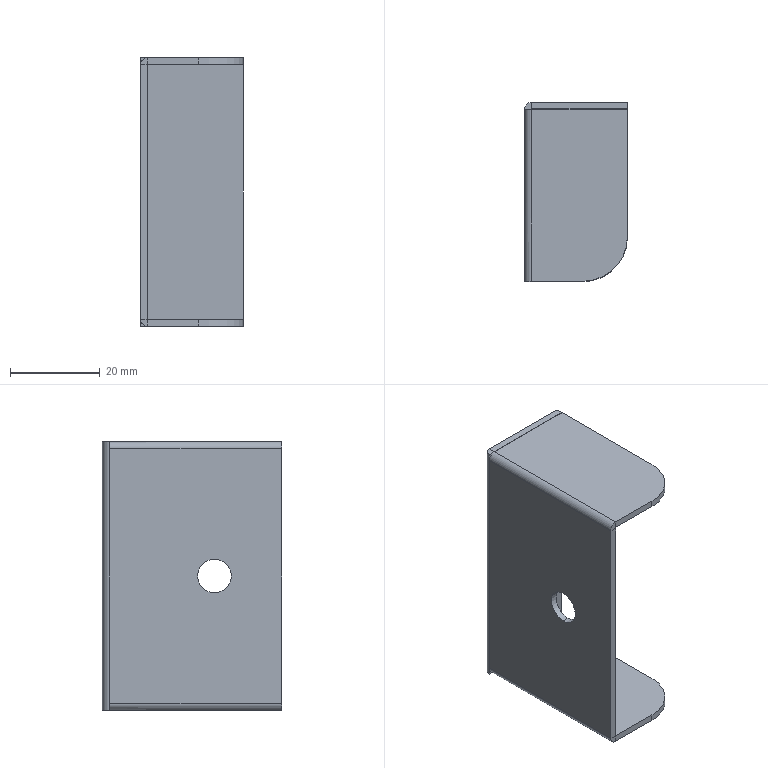Component | SolidWorks | TopPlateWelding-1_AxisFixingPlate2-1 | 1 solid | 37 faces | box 23 x 40 x 60 mm | volume 7806 mm3 | plane 27 | cylinder 10 | commonest cylinder face diameters 0.2 x3 3.2 x3 7.5 x2 20 x2
STEP:
#1=COLOUR_RGB('',0.7922,0.8196,0.9333);
#2=FILL_AREA_STYLE_COLOUR('',#1);
#3=FILL_AREA_STYLE('',(#2));
#4=SURFACE_STYLE_FILL_AREA(#3);
#5=SURFACE_SIDE_STYLE('',(#4));
#6=SURFACE_STYLE_USAGE(.BOTH.,#5);
#7=PRESENTATION_STYLE_ASSIGNMENT((#6));
#8=CARTESIAN_POINT('',(8.937,5.032,15.128));
#9=VERTEX_POINT('',#8);
#10=CARTESIAN_POINT('',(8.937,5.032,14.833));
#11=VERTEX_POINT('',#10);
#12=CARTESIAN_POINT('',(8.937,5.032,14.98));
#13=DIRECTION('',(-1.,-0.,0.));
#14=DIRECTION('',(0.,-1.,0.));
#15=AXIS2_PLACEMENT_3D('',#12,#13,#14);
#16=CIRCLE('',#15,0.1476);
#17=EDGE_CURVE('',#9,#11,#16,.T.);
#18=ORIENTED_EDGE('',*,*,#17,.F.);
#19=CARTESIAN_POINT('',(8.878,5.032,15.128));
#20=VERTEX_POINT('',#19);
#21=CARTESIAN_POINT('',(9.355,5.032,15.128));
#22=DIRECTION('',(-1.,-0.,0.));
#23=VECTOR('',#22,39.37);
#24=LINE('',#21,#23);
#25=EDGE_CURVE('',#9,#20,#24,.T.);
#26=ORIENTED_EDGE('',*,*,#25,.T.);
#27=CARTESIAN_POINT('',(8.878,5.032,14.833));
#28=VERTEX_POINT('',#27);
#29=CARTESIAN_POINT('',(8.878,5.032,14.98));
#30=DIRECTION('',(-1.,-0.,0.));
#31=DIRECTION('',(-0.,0.,-1.));
#32=AXIS2_PLACEMENT_3D('',#29,#30,#31);
#33=CIRCLE('',#32,0.1476);
#34=EDGE_CURVE('',#20,#28,#33,.T.);
#35=ORIENTED_EDGE('',*,*,#34,.T.);
#36=CARTESIAN_POINT('',(9.355,5.032,14.833));
#37=DIRECTION('',(-1.,-0.,0.));
#38=VECTOR('',#37,39.37);
#39=LINE('',#36,#38);
#40=EDGE_CURVE('',#11,#28,#39,.T.);
#41=ORIENTED_EDGE('',*,*,#40,.F.);
#42=EDGE_LOOP('',(#18,#26,#35,#41));
#43=FACE_OUTER_BOUND('',#42,.T.);
#44=CARTESIAN_POINT('',(9.355,5.032,14.98));
#45=DIRECTION('',(-1.,-0.,0.));
#46=DIRECTION('',(-0.,0.,-1.));
#47=AXIS2_PLACEMENT_3D('',#44,#45,#46);
#48=CYLINDRICAL_SURFACE('',#47,0.1476);
#49=ADVANCED_FACE('',(#43),#48,.F.);
#50=CARTESIAN_POINT('',(8.878,5.954,16.161));
#51=VERTEX_POINT('',#50);
#52=CARTESIAN_POINT('',(8.878,5.954,16.098));
#53=VERTEX_POINT('',#52);
#54=CARTESIAN_POINT('',(8.878,5.954,13.799));
#55=DIRECTION('',(-0.,-0.,-1.));
#56=VECTOR('',#55,39.37);
#57=LINE('',#54,#56);
#58=EDGE_CURVE('',#51,#53,#57,.T.);
#59=ORIENTED_EDGE('',*,*,#58,.T.);
#60=CARTESIAN_POINT('',(8.937,5.954,16.161));
#61=VERTEX_POINT('',#60);
#62=CARTESIAN_POINT('',(8.941,5.954,16.098));
#63=DIRECTION('',(-0.,1.,-0.));
#64=DIRECTION('',(0.,0.,-1.));
#65=AXIS2_PLACEMENT_3D('',#62,#63,#64);
#66=CIRCLE('',#65,0.06299);
#67=EDGE_CURVE('',#53,#61,#66,.T.);
#68=ORIENTED_EDGE('',*,*,#67,.T.);
#69=CARTESIAN_POINT('',(8.937,5.954,16.161));
#70=VERTEX_POINT('',#69);
#71=CARTESIAN_POINT('',(8.937,5.954,16.098));
#72=DIRECTION('',(0.,-0.,1.));
#73=VECTOR('',#72,39.37);
#74=LINE('',#71,#73);
#75=EDGE_CURVE('',#61,#70,#74,.T.);
#76=ORIENTED_EDGE('',*,*,#75,.T.);
#77=CARTESIAN_POINT('',(8.937,5.954,16.161));
#78=DIRECTION('',(-1.,-0.,0.));
#79=VECTOR('',#78,39.37);
#80=LINE('',#77,#79);
#81=EDGE_CURVE('',#70,#51,#80,.T.);
#82=ORIENTED_EDGE('',*,*,#81,.T.);
#83=EDGE_LOOP('',(#59,#68,#76,#82));
#84=FACE_OUTER_BOUND('',#83,.T.);
#85=CARTESIAN_POINT('',(8.937,5.954,16.098));
#86=DIRECTION('',(0.,-1.,-0.));
#87=DIRECTION('',(-0.,0.,-1.));
#88=AXIS2_PLACEMENT_3D('',#85,#86,#87);
#89=PLANE('',#88);
#90=ADVANCED_FACE('',(#84),#89,.T.);
#91=CARTESIAN_POINT('',(8.937,5.032,14.98));
#92=DIRECTION('',(-1.,-0.,0.));
#93=DIRECTION('',(0.,-1.,0.));
#94=AXIS2_PLACEMENT_3D('',#91,#92,#93);
#95=CIRCLE('',#94,0.1476);
#96=EDGE_CURVE('',#11,#9,#95,.T.);
#97=ORIENTED_EDGE('',*,*,#96,.T.);
#98=ORIENTED_EDGE('',*,*,#17,.T.);
#99=EDGE_LOOP('',(#97,#98));
#100=FACE_BOUND('',#99,.T.);
#101=CARTESIAN_POINT('',(8.937,5.954,13.862));
#102=VERTEX_POINT('',#101);
#103=CARTESIAN_POINT('',(8.937,5.954,16.098));
#104=VERTEX_POINT('',#103);
#105=CARTESIAN_POINT('',(8.937,5.954,13.799));
#106=DIRECTION('',(0.,0.,1.));
#107=VECTOR('',#106,39.37);
#108=LINE('',#105,#107);
#109=EDGE_CURVE('',#102,#104,#108,.T.);
#110=ORIENTED_EDGE('',*,*,#109,.T.);
#111=CARTESIAN_POINT('',(8.937,4.442,16.098));
#112=VERTEX_POINT('',#111);
#113=CARTESIAN_POINT('',(8.937,4.442,16.098));
#114=DIRECTION('',(-0.,1.,-0.));
#115=VECTOR('',#114,39.37);
#116=LINE('',#113,#115);
#117=EDGE_CURVE('',#112,#104,#116,.T.);
#118=ORIENTED_EDGE('',*,*,#117,.F.);
#119=CARTESIAN_POINT('',(8.937,4.442,13.862));
#120=VERTEX_POINT('',#119);
#121=CARTESIAN_POINT('',(8.937,4.442,13.799));
#122=DIRECTION('',(0.,0.,1.));
#123=VECTOR('',#122,39.37);
#124=LINE('',#121,#123);
#125=EDGE_CURVE('',#120,#112,#124,.T.);
#126=ORIENTED_EDGE('',*,*,#125,.F.);
#127=CARTESIAN_POINT('',(8.937,5.954,13.862));
#128=DIRECTION('',(0.,-1.,0.));
#129=VECTOR('',#128,39.37);
#130=LINE('',#127,#129);
#131=EDGE_CURVE('',#102,#120,#130,.T.);
#132=ORIENTED_EDGE('',*,*,#131,.F.);
#133=EDGE_LOOP('',(#110,#118,#126,#132));
#134=FACE_OUTER_BOUND('',#133,.T.);
#135=CARTESIAN_POINT('',(8.937,4.442,13.799));
#136=DIRECTION('',(1.,0.,-0.));
#137=DIRECTION('',(0.,-1.,0.));
#138=AXIS2_PLACEMENT_3D('',#135,#136,#137);
#139=PLANE('',#138);
#140=ADVANCED_FACE('',(#100,#134),#139,.T.);
#141=CARTESIAN_POINT('',(8.878,5.032,14.98));
#142=DIRECTION('',(-1.,-0.,0.));
#143=DIRECTION('',(-0.,0.,-1.));
#144=AXIS2_PLACEMENT_3D('',#141,#142,#143);
#145=CIRCLE('',#144,0.1476);
#146=EDGE_CURVE('',#28,#20,#145,.T.);
#147=ORIENTED_EDGE('',*,*,#146,.F.);
#148=ORIENTED_EDGE('',*,*,#34,.F.);
#149=EDGE_LOOP('',(#147,#148));
#150=FACE_BOUND('',#149,.T.);
#151=CARTESIAN_POINT('',(8.878,4.442,16.098));
#152=VERTEX_POINT('',#151);
#153=CARTESIAN_POINT('',(8.878,4.442,16.098));
#154=DIRECTION('',(-0.,1.,-0.));
#155=VECTOR('',#154,39.37);
#156=LINE('',#153,#155);
#157=EDGE_CURVE('',#152,#53,#156,.T.);
#158=ORIENTED_EDGE('',*,*,#157,.T.);
#159=CARTESIAN_POINT('',(8.878,5.954,13.862));
#160=VERTEX_POINT('',#159);
#161=CARTESIAN_POINT('',(8.878,5.954,13.799));
#162=DIRECTION('',(0.,0.,1.));
#163=VECTOR('',#162,39.37);
#164=LINE('',#161,#163);
#165=EDGE_CURVE('',#160,#53,#164,.T.);
#166=ORIENTED_EDGE('',*,*,#165,.F.);
#167=CARTESIAN_POINT('',(8.878,4.442,13.862));
#168=VERTEX_POINT('',#167);
#169=CARTESIAN_POINT('',(8.878,5.954,13.862));
#170=DIRECTION('',(0.,-1.,0.));
#171=VECTOR('',#170,39.37);
#172=LINE('',#169,#171);
#173=EDGE_CURVE('',#160,#168,#172,.T.);
#174=ORIENTED_EDGE('',*,*,#173,.T.);
#175=CARTESIAN_POINT('',(8.878,4.442,13.799));
#176=DIRECTION('',(0.,0.,1.));
#177=VECTOR('',#176,39.37);
#178=LINE('',#175,#177);
#179=EDGE_CURVE('',#168,#152,#178,.T.);
#180=ORIENTED_EDGE('',*,*,#179,.T.);
#181=EDGE_LOOP('',(#158,#166,#174,#180));
#182=FACE_OUTER_BOUND('',#181,.T.);
#183=CARTESIAN_POINT('',(8.878,4.442,13.799));
#184=DIRECTION('',(1.,0.,-0.));
#185=DIRECTION('',(0.,-1.,0.));
#186=AXIS2_PLACEMENT_3D('',#183,#184,#185);
#187=PLANE('',#186);
#188=ADVANCED_FACE('',(#150,#182),#187,.F.);
#189=ORIENTED_EDGE('',*,*,#125,.T.);
#190=CARTESIAN_POINT('',(8.937,4.442,16.098));
#191=DIRECTION('',(-1.,-0.,0.));
#192=VECTOR('',#191,39.37);
#193=LINE('',#190,#192);
#194=EDGE_CURVE('',#112,#152,#193,.T.);
#195=ORIENTED_EDGE('',*,*,#194,.T.);
#196=ORIENTED_EDGE('',*,*,#179,.F.);
#197=CARTESIAN_POINT('',(8.937,4.442,13.862));
#198=DIRECTION('',(-1.,-0.,0.));
#199=VECTOR('',#198,39.37);
#200=LINE('',#197,#199);
#201=EDGE_CURVE('',#120,#168,#200,.T.);
#202=ORIENTED_EDGE('',*,*,#201,.F.);
#203=EDGE_LOOP('',(#189,#195,#196,#202));
#204=FACE_OUTER_BOUND('',#203,.T.);
#205=CARTESIAN_POINT('',(8.878,4.442,13.799));
#206=DIRECTION('',(0.,-1.,0.));
#207=DIRECTION('',(-0.,-0.,-1.));
#208=AXIS2_PLACEMENT_3D('',#205,#206,#207);
#209=PLANE('',#208);
#210=ADVANCED_FACE('',(#204),#209,.T.);
#211=CARTESIAN_POINT('',(8.937,5.954,13.799));
#212=VERTEX_POINT('',#211);
#213=CARTESIAN_POINT('',(8.937,5.954,13.799));
#214=VERTEX_POINT('',#213);
#215=CARTESIAN_POINT('',(8.937,5.954,13.799));
#216=DIRECTION('',(0.,0.,1.));
#217=VECTOR('',#216,39.37);
#218=LINE('',#215,#217);
#219=EDGE_CURVE('',#212,#214,#218,.T.);
#220=ORIENTED_EDGE('',*,*,#219,.T.);
#221=CARTESIAN_POINT('',(8.941,5.954,13.862));
#222=DIRECTION('',(-0.,1.,-0.));
#223=DIRECTION('',(0.,0.,1.));
#224=AXIS2_PLACEMENT_3D('',#221,#222,#223);
#225=CIRCLE('',#224,0.06299);
#226=EDGE_CURVE('',#214,#160,#225,.T.);
#227=ORIENTED_EDGE('',*,*,#226,.T.);
#228=CARTESIAN_POINT('',(8.878,5.954,13.799));
#229=VERTEX_POINT('',#228);
#230=CARTESIAN_POINT('',(8.878,5.954,13.799));
#231=DIRECTION('',(0.,0.,1.));
#232=VECTOR('',#231,39.37);
#233=LINE('',#230,#232);
#234=EDGE_CURVE('',#229,#160,#233,.T.);
#235=ORIENTED_EDGE('',*,*,#234,.F.);
#236=CARTESIAN_POINT('',(8.878,5.954,13.799));
#237=DIRECTION('',(1.,0.,-0.));
#238=VECTOR('',#237,39.37);
#239=LINE('',#236,#238);
#240=EDGE_CURVE('',#229,#212,#239,.T.);
#241=ORIENTED_EDGE('',*,*,#240,.T.);
#242=EDGE_LOOP('',(#220,#227,#235,#241));
#243=FACE_OUTER_BOUND('',#242,.T.);
#244=CARTESIAN_POINT('',(8.937,5.954,13.799));
#245=DIRECTION('',(0.,-1.,0.));
#246=DIRECTION('',(-0.,-0.,-1.));
#247=AXIS2_PLACEMENT_3D('',#244,#245,#246);
#248=PLANE('',#247);
#249=ADVANCED_FACE('',(#243),#248,.T.);
#250=ORIENTED_EDGE('',*,*,#240,.F.);
#251=CARTESIAN_POINT('',(8.941,6.017,13.799));
#252=VERTEX_POINT('',#251);
#253=CARTESIAN_POINT('',(8.941,5.954,13.799));
#254=DIRECTION('',(-0.,-0.,-1.));
#255=DIRECTION('',(-1.,0.,0.));
#256=AXIS2_PLACEMENT_3D('',#253,#254,#255);
#257=CIRCLE('',#256,0.06299);
#258=EDGE_CURVE('',#229,#252,#257,.T.);
#259=ORIENTED_EDGE('',*,*,#258,.T.);
#260=CARTESIAN_POINT('',(8.941,5.958,13.799));
#261=VERTEX_POINT('',#260);
#262=CARTESIAN_POINT('',(8.941,5.958,13.799));
#263=DIRECTION('',(-0.,1.,-0.));
#264=VECTOR('',#263,39.37);
#265=LINE('',#262,#264);
#266=EDGE_CURVE('',#261,#252,#265,.T.);
#267=ORIENTED_EDGE('',*,*,#266,.F.);
#268=CARTESIAN_POINT('',(8.941,5.954,13.799));
#269=DIRECTION('',(-0.,-0.,-1.));
#270=DIRECTION('',(1.,0.,0.));
#271=AXIS2_PLACEMENT_3D('',#268,#269,#270);
#272=CIRCLE('',#271,0.003937);
#273=EDGE_CURVE('',#212,#261,#272,.T.);
#274=ORIENTED_EDGE('',*,*,#273,.F.);
#275=EDGE_LOOP('',(#250,#259,#267,#274));
#276=FACE_OUTER_BOUND('',#275,.T.);
#277=CARTESIAN_POINT('',(8.878,5.954,13.799));
#278=DIRECTION('',(-0.,-0.,-1.));
#279=DIRECTION('',(1.,0.,-0.));
#280=AXIS2_PLACEMENT_3D('',#277,#278,#279);
#281=PLANE('',#280);
#282=ADVANCED_FACE('',(#276),#281,.T.);
#283=CARTESIAN_POINT('',(8.941,6.017,16.161));
#284=VERTEX_POINT('',#283);
#285=CARTESIAN_POINT('',(8.941,5.958,16.161));
#286=VERTEX_POINT('',#285);
#287=CARTESIAN_POINT('',(8.941,6.017,16.161));
#288=DIRECTION('',(0.,-1.,0.));
#289=VECTOR('',#288,39.37);
#290=LINE('',#287,#289);
#291=EDGE_CURVE('',#284,#286,#290,.T.);
#292=ORIENTED_EDGE('',*,*,#291,.F.);
#293=CARTESIAN_POINT('',(8.941,5.954,16.161));
#294=DIRECTION('',(-0.,-0.,-1.));
#295=DIRECTION('',(-1.,0.,0.));
#296=AXIS2_PLACEMENT_3D('',#293,#294,#295);
#297=CIRCLE('',#296,0.06299);
#298=EDGE_CURVE('',#51,#284,#297,.T.);
#299=ORIENTED_EDGE('',*,*,#298,.F.);
#300=ORIENTED_EDGE('',*,*,#81,.F.);
#301=CARTESIAN_POINT('',(8.941,5.954,16.161));
#302=DIRECTION('',(-0.,-0.,-1.));
#303=DIRECTION('',(1.,0.,0.));
#304=AXIS2_PLACEMENT_3D('',#301,#302,#303);
#305=CIRCLE('',#304,0.003937);
#306=EDGE_CURVE('',#70,#286,#305,.T.);
#307=ORIENTED_EDGE('',*,*,#306,.T.);
#308=EDGE_LOOP('',(#292,#299,#300,#307));
#309=FACE_OUTER_BOUND('',#308,.T.);
#310=CARTESIAN_POINT('',(8.941,6.017,16.161));
#311=DIRECTION('',(0.,0.,1.));
#312=DIRECTION('',(-1.,-0.,0.));
#313=AXIS2_PLACEMENT_3D('',#310,#311,#312);
#314=PLANE('',#313);
#315=ADVANCED_FACE('',(#309),#314,.T.);
#316=CARTESIAN_POINT('',(9.783,5.958,16.161));
#317=VERTEX_POINT('',#316);
#318=CARTESIAN_POINT('',(9.783,6.011,16.161));
#319=VERTEX_POINT('',#318);
#320=CARTESIAN_POINT('',(9.783,5.958,16.161));
#321=DIRECTION('',(-0.,1.,-0.));
#322=VECTOR('',#321,39.37);
#323=LINE('',#320,#322);
#324=EDGE_CURVE('',#317,#319,#323,.T.);
#325=ORIENTED_EDGE('',*,*,#324,.T.);
#326=CARTESIAN_POINT('',(9.778,6.017,16.161));
#327=VERTEX_POINT('',#326);
#328=CARTESIAN_POINT('',(9.389,6.405,16.161));
#329=DIRECTION('',(-0.7071,0.7071,0.));
#330=VECTOR('',#329,39.37);
#331=LINE('',#328,#330);
#332=EDGE_CURVE('',#319,#327,#331,.T.);
#333=ORIENTED_EDGE('',*,*,#332,.T.);
#334=CARTESIAN_POINT('',(8.878,6.017,16.161));
#335=DIRECTION('',(1.,0.,-0.));
#336=VECTOR('',#335,39.37);
#337=LINE('',#334,#336);
#338=EDGE_CURVE('',#284,#327,#337,.T.);
#339=ORIENTED_EDGE('',*,*,#338,.F.);
#340=ORIENTED_EDGE('',*,*,#291,.T.);
#341=CARTESIAN_POINT('',(8.878,5.958,16.161));
#342=DIRECTION('',(1.,0.,-0.));
#343=VECTOR('',#342,39.37);
#344=LINE('',#341,#343);
#345=EDGE_CURVE('',#286,#317,#344,.T.);
#346=ORIENTED_EDGE('',*,*,#345,.T.);
#347=EDGE_LOOP('',(#325,#333,#339,#340,#346));
#348=FACE_OUTER_BOUND('',#347,.T.);
#349=CARTESIAN_POINT('',(8.937,5.954,16.161));
#350=DIRECTION('',(0.,0.,1.));
#351=DIRECTION('',(-1.,-0.,0.));
#352=AXIS2_PLACEMENT_3D('',#349,#350,#351);
#353=PLANE('',#352);
#354=ADVANCED_FACE('',(#348),#353,.T.);
#355=ORIENTED_EDGE('',*,*,#338,.T.);
#356=CARTESIAN_POINT('',(9.778,6.017,13.799));
#357=VERTEX_POINT('',#356);
#358=CARTESIAN_POINT('',(9.778,6.017,13.799));
#359=DIRECTION('',(-0.,-0.,-1.));
#360=VECTOR('',#359,39.37);
#361=LINE('',#358,#360);
#362=EDGE_CURVE('',#327,#357,#361,.T.);
#363=ORIENTED_EDGE('',*,*,#362,.T.);
#364=CARTESIAN_POINT('',(8.878,6.017,13.799));
#365=DIRECTION('',(1.,0.,-0.));
#366=VECTOR('',#365,39.37);
#367=LINE('',#364,#366);
#368=EDGE_CURVE('',#252,#357,#367,.T.);
#369=ORIENTED_EDGE('',*,*,#368,.F.);
#370=CARTESIAN_POINT('',(8.941,6.017,13.799));
#371=DIRECTION('',(0.,0.,1.));
#372=VECTOR('',#371,39.37);
#373=LINE('',#370,#372);
#374=EDGE_CURVE('',#252,#284,#373,.T.);
#375=ORIENTED_EDGE('',*,*,#374,.T.);
#376=EDGE_LOOP('',(#355,#363,#369,#375));
#377=FACE_OUTER_BOUND('',#376,.T.);
#378=CARTESIAN_POINT('',(8.878,6.017,13.799));
#379=DIRECTION('',(0.,-1.,0.));
#380=DIRECTION('',(-0.,-0.,-1.));
#381=AXIS2_PLACEMENT_3D('',#378,#379,#380);
#382=PLANE('',#381);
#383=ADVANCED_FACE('',(#377),#382,.F.);
#384=CARTESIAN_POINT('',(9.783,5.958,13.799));
#385=VERTEX_POINT('',#384);
#386=CARTESIAN_POINT('',(9.783,6.011,13.799));
#387=VERTEX_POINT('',#386);
#388=CARTESIAN_POINT('',(9.783,5.958,13.799));
#389=DIRECTION('',(-0.,1.,-0.));
#390=VECTOR('',#389,39.37);
#391=LINE('',#388,#390);
#392=EDGE_CURVE('',#385,#387,#391,.T.);
#393=ORIENTED_EDGE('',*,*,#392,.T.);
#394=CARTESIAN_POINT('',(9.783,6.011,16.161));
#395=DIRECTION('',(0.,0.,1.));
#396=VECTOR('',#395,39.37);
#397=LINE('',#394,#396);
#398=EDGE_CURVE('',#387,#319,#397,.T.);
#399=ORIENTED_EDGE('',*,*,#398,.T.);
#400=ORIENTED_EDGE('',*,*,#324,.F.);
#401=CARTESIAN_POINT('',(9.783,5.958,13.799));
#402=DIRECTION('',(0.,0.,1.));
#403=VECTOR('',#402,39.37);
#404=LINE('',#401,#403);
#405=EDGE_CURVE('',#385,#317,#404,.T.);
#406=ORIENTED_EDGE('',*,*,#405,.F.);
#407=EDGE_LOOP('',(#393,#399,#400,#406));
#408=FACE_OUTER_BOUND('',#407,.T.);
#409=CARTESIAN_POINT('',(9.783,5.958,13.799));
#410=DIRECTION('',(1.,0.,-0.));
#411=DIRECTION('',(0.,0.,1.));
#412=AXIS2_PLACEMENT_3D('',#409,#410,#411);
#413=PLANE('',#412);
#414=ADVANCED_FACE('',(#408),#413,.T.);
#415=ORIENTED_EDGE('',*,*,#345,.F.);
#416=CARTESIAN_POINT('',(8.941,5.958,13.799));
#417=DIRECTION('',(0.,0.,1.));
#418=VECTOR('',#417,39.37);
#419=LINE('',#416,#418);
#420=EDGE_CURVE('',#261,#286,#419,.T.);
#421=ORIENTED_EDGE('',*,*,#420,.F.);
#422=CARTESIAN_POINT('',(8.878,5.958,13.799));
#423=DIRECTION('',(1.,0.,-0.));
#424=VECTOR('',#423,39.37);
#425=LINE('',#422,#424);
#426=EDGE_CURVE('',#261,#385,#425,.T.);
#427=ORIENTED_EDGE('',*,*,#426,.T.);
#428=ORIENTED_EDGE('',*,*,#405,.T.);
#429=EDGE_LOOP('',(#415,#421,#427,#428));
#430=FACE_OUTER_BOUND('',#429,.T.);
#431=CARTESIAN_POINT('',(8.878,5.958,13.799));
#432=DIRECTION('',(0.,-1.,0.));
#433=DIRECTION('',(-0.,-0.,-1.));
#434=AXIS2_PLACEMENT_3D('',#431,#432,#433);
#435=PLANE('',#434);
#436=ADVANCED_FACE('',(#430),#435,.T.);
#437=ORIENTED_EDGE('',*,*,#306,.F.);
#438=ORIENTED_EDGE('',*,*,#75,.F.);
#439=CARTESIAN_POINT('',(8.937,5.954,16.098));
#440=DIRECTION('',(0.,-0.,1.));
#441=VECTOR('',#440,39.37);
#442=LINE('',#439,#441);
#443=EDGE_CURVE('',#104,#61,#442,.T.);
#444=ORIENTED_EDGE('',*,*,#443,.F.);
#445=ORIENTED_EDGE('',*,*,#109,.F.);
#446=CARTESIAN_POINT('',(8.937,5.954,13.799));
#447=DIRECTION('',(0.,0.,1.));
#448=VECTOR('',#447,39.37);
#449=LINE('',#446,#448);
#450=EDGE_CURVE('',#214,#102,#449,.T.);
#451=ORIENTED_EDGE('',*,*,#450,.F.);
#452=ORIENTED_EDGE('',*,*,#219,.F.);
#453=ORIENTED_EDGE('',*,*,#273,.T.);
#454=ORIENTED_EDGE('',*,*,#420,.T.);
#455=EDGE_LOOP('',(#437,#438,#444,#445,#451,#452,#453,#454));
#456=FACE_OUTER_BOUND('',#455,.T.);
#457=CARTESIAN_POINT('',(8.941,5.954,13.799));
#458=DIRECTION('',(0.,0.,1.));
#459=DIRECTION('',(-1.,0.,0.));
#460=AXIS2_PLACEMENT_3D('',#457,#458,#459);
#461=CYLINDRICAL_SURFACE('',#460,0.003937);
#462=ADVANCED_FACE('',(#456),#461,.F.);
#463=ORIENTED_EDGE('',*,*,#298,.T.);
#464=ORIENTED_EDGE('',*,*,#374,.F.);
#465=ORIENTED_EDGE('',*,*,#258,.F.);
#466=ORIENTED_EDGE('',*,*,#234,.T.);
#467=ORIENTED_EDGE('',*,*,#165,.T.);
#468=ORIENTED_EDGE('',*,*,#58,.F.);
#469=EDGE_LOOP('',(#463,#464,#465,#466,#467,#468));
#470=FACE_OUTER_BOUND('',#469,.T.);
#471=CARTESIAN_POINT('',(8.941,5.954,13.799));
#472=DIRECTION('',(0.,0.,1.));
#473=DIRECTION('',(-1.,0.,0.));
#474=AXIS2_PLACEMENT_3D('',#471,#472,#473);
#475=CYLINDRICAL_SURFACE('',#474,0.06299);
#476=ADVANCED_FACE('',(#470),#475,.T.);
#477=ORIENTED_EDGE('',*,*,#368,.T.);
#478=CARTESIAN_POINT('',(9.391,6.403,13.799));
#479=DIRECTION('',(0.7071,-0.7071,-0.));
#480=VECTOR('',#479,39.37);
#481=LINE('',#478,#480);
#482=EDGE_CURVE('',#357,#387,#481,.T.);
#483=ORIENTED_EDGE('',*,*,#482,.T.);
#484=ORIENTED_EDGE('',*,*,#392,.F.);
#485=ORIENTED_EDGE('',*,*,#426,.F.);
#486=ORIENTED_EDGE('',*,*,#266,.T.);
#487=EDGE_LOOP('',(#477,#483,#484,#485,#486));
#488=FACE_OUTER_BOUND('',#487,.T.);
#489=CARTESIAN_POINT('',(8.941,5.954,13.799));
#490=DIRECTION('',(-0.,-0.,-1.));
#491=DIRECTION('',(1.,0.,-0.));
#492=AXIS2_PLACEMENT_3D('',#489,#490,#491);
#493=PLANE('',#492);
#494=ADVANCED_FACE('',(#488),#493,.T.);
#495=ORIENTED_EDGE('',*,*,#25,.F.);
#496=ORIENTED_EDGE('',*,*,#96,.F.);
#497=ORIENTED_EDGE('',*,*,#40,.T.);
#498=ORIENTED_EDGE('',*,*,#146,.T.);
#499=EDGE_LOOP('',(#495,#496,#497,#498));
#500=FACE_OUTER_BOUND('',#499,.T.);
#501=CARTESIAN_POINT('',(9.355,5.032,14.98));
#502=DIRECTION('',(-1.,-0.,0.));
#503=DIRECTION('',(-0.,0.,-1.));
#504=AXIS2_PLACEMENT_3D('',#501,#502,#503);
#505=CYLINDRICAL_SURFACE('',#504,0.1476);
#506=ADVANCED_FACE('',(#500),#505,.F.);
#507=CARTESIAN_POINT('',(8.941,4.442,13.858));
#508=VERTEX_POINT('',#507);
#509=CARTESIAN_POINT('',(8.941,4.442,13.799));
#510=VERTEX_POINT('',#509);
#511=CARTESIAN_POINT('',(8.941,4.442,13.799));
#512=DIRECTION('',(-0.,-0.,-1.));
#513=VECTOR('',#512,39.37);
#514=LINE('',#511,#513);
#515=EDGE_CURVE('',#508,#510,#514,.T.);
#516=ORIENTED_EDGE('',*,*,#515,.F.);
#517=CARTESIAN_POINT('',(8.941,4.442,13.862));
#518=DIRECTION('',(0.,-1.,0.));
#519=DIRECTION('',(0.,0.,1.));
#520=AXIS2_PLACEMENT_3D('',#517,#518,#519);
#521=CIRCLE('',#520,0.003937);
#522=EDGE_CURVE('',#120,#508,#521,.T.);
#523=ORIENTED_EDGE('',*,*,#522,.F.);
#524=ORIENTED_EDGE('',*,*,#201,.T.);
#525=CARTESIAN_POINT('',(8.941,4.442,13.862));
#526=DIRECTION('',(0.,-1.,0.));
#527=DIRECTION('',(0.,0.,1.));
#528=AXIS2_PLACEMENT_3D('',#525,#526,#527);
#529=CIRCLE('',#528,0.06299);
#530=EDGE_CURVE('',#168,#510,#529,.T.);
#531=ORIENTED_EDGE('',*,*,#530,.T.);
#532=EDGE_LOOP('',(#516,#523,#524,#531));
#533=FACE_OUTER_BOUND('',#532,.T.);
#534=CARTESIAN_POINT('',(8.941,4.442,13.862));
#535=DIRECTION('',(0.,-1.,0.));
#536=DIRECTION('',(-0.,-0.,-1.));
#537=AXIS2_PLACEMENT_3D('',#534,#535,#536);
#538=PLANE('',#537);
#539=ADVANCED_FACE('',(#533),#538,.T.);
#540=CARTESIAN_POINT('',(8.941,5.954,13.799));
#541=VERTEX_POINT('',#540);
#542=CARTESIAN_POINT('',(8.941,5.954,13.862));
#543=DIRECTION('',(-0.,1.,-0.));
#544=DIRECTION('',(0.,0.,1.));
#545=AXIS2_PLACEMENT_3D('',#542,#543,#544);
#546=CIRCLE('',#545,0.06299);
#547=EDGE_CURVE('',#541,#214,#546,.T.);
#548=ORIENTED_EDGE('',*,*,#547,.T.);
#549=ORIENTED_EDGE('',*,*,#450,.T.);
#550=CARTESIAN_POINT('',(8.941,5.954,13.858));
#551=VERTEX_POINT('',#550);
#552=CARTESIAN_POINT('',(8.941,5.954,13.862));
#553=DIRECTION('',(-0.,1.,-0.));
#554=DIRECTION('',(0.,0.,1.));
#555=AXIS2_PLACEMENT_3D('',#552,#553,#554);
#556=CIRCLE('',#555,0.003937);
#557=EDGE_CURVE('',#551,#102,#556,.T.);
#558=ORIENTED_EDGE('',*,*,#557,.F.);
#559=CARTESIAN_POINT('',(8.941,5.954,13.858));
#560=DIRECTION('',(-0.,-0.,-1.));
#561=VECTOR('',#560,39.37);
#562=LINE('',#559,#561);
#563=EDGE_CURVE('',#551,#541,#562,.T.);
#564=ORIENTED_EDGE('',*,*,#563,.T.);
#565=EDGE_LOOP('',(#548,#549,#558,#564));
#566=FACE_OUTER_BOUND('',#565,.T.);
#567=CARTESIAN_POINT('',(8.941,5.954,13.862));
#568=DIRECTION('',(0.,-1.,0.));
#569=DIRECTION('',(-0.,-0.,-1.));
#570=AXIS2_PLACEMENT_3D('',#567,#568,#569);
#571=PLANE('',#570);
#572=ADVANCED_FACE('',(#566),#571,.F.);
#573=ORIENTED_EDGE('',*,*,#173,.F.);
#574=ORIENTED_EDGE('',*,*,#226,.F.);
#575=ORIENTED_EDGE('',*,*,#547,.F.);
#576=CARTESIAN_POINT('',(8.941,6.017,13.799));
#577=DIRECTION('',(-0.,1.,-0.));
#578=VECTOR('',#577,39.37);
#579=LINE('',#576,#578);
#580=EDGE_CURVE('',#510,#541,#579,.T.);
#581=ORIENTED_EDGE('',*,*,#580,.F.);
#582=ORIENTED_EDGE('',*,*,#530,.F.);
#583=EDGE_LOOP('',(#573,#574,#575,#581,#582));
#584=FACE_OUTER_BOUND('',#583,.T.);
#585=CARTESIAN_POINT('',(8.941,5.954,13.862));
#586=DIRECTION('',(-0.,1.,-0.));
#587=DIRECTION('',(0.,0.,-1.));
#588=AXIS2_PLACEMENT_3D('',#585,#586,#587);
#589=CYLINDRICAL_SURFACE('',#588,0.06299);
#590=ADVANCED_FACE('',(#584),#589,.T.);
#591=ORIENTED_EDGE('',*,*,#131,.T.);
#592=ORIENTED_EDGE('',*,*,#522,.T.);
#593=CARTESIAN_POINT('',(8.941,4.442,13.858));
#594=DIRECTION('',(-0.,1.,-0.));
#595=VECTOR('',#594,39.37);
#596=LINE('',#593,#595);
#597=EDGE_CURVE('',#508,#551,#596,.T.);
#598=ORIENTED_EDGE('',*,*,#597,.T.);
#599=ORIENTED_EDGE('',*,*,#557,.T.);
#600=EDGE_LOOP('',(#591,#592,#598,#599));
#601=FACE_OUTER_BOUND('',#600,.T.);
#602=CARTESIAN_POINT('',(8.941,5.954,13.862));
#603=DIRECTION('',(-0.,1.,-0.));
#604=DIRECTION('',(0.,0.,-1.));
#605=AXIS2_PLACEMENT_3D('',#602,#603,#604);
#606=CYLINDRICAL_SURFACE('',#605,0.003937);
#607=ADVANCED_FACE('',(#601),#606,.F.);
#608=CARTESIAN_POINT('',(9.39,4.442,13.799));
#609=VERTEX_POINT('',#608);
#610=CARTESIAN_POINT('',(8.878,4.442,13.799));
#611=DIRECTION('',(-1.,-0.,0.));
#612=VECTOR('',#611,39.37);
#613=LINE('',#610,#612);
#614=EDGE_CURVE('',#609,#510,#613,.T.);
#615=ORIENTED_EDGE('',*,*,#614,.F.);
#616=CARTESIAN_POINT('',(9.39,4.442,13.858));
#617=VERTEX_POINT('',#616);
#618=CARTESIAN_POINT('',(9.39,4.442,13.799));
#619=DIRECTION('',(0.,0.,1.));
#620=VECTOR('',#619,39.37);
#621=LINE('',#618,#620);
#622=EDGE_CURVE('',#609,#617,#621,.T.);
#623=ORIENTED_EDGE('',*,*,#622,.T.);
#624=CARTESIAN_POINT('',(8.937,4.442,13.858));
#625=DIRECTION('',(-1.,-0.,0.));
#626=VECTOR('',#625,39.37);
#627=LINE('',#624,#626);
#628=EDGE_CURVE('',#617,#508,#627,.T.);
#629=ORIENTED_EDGE('',*,*,#628,.T.);
#630=ORIENTED_EDGE('',*,*,#515,.T.);
#631=EDGE_LOOP('',(#615,#623,#629,#630));
#632=FACE_OUTER_BOUND('',#631,.T.);
#633=CARTESIAN_POINT('',(8.937,4.442,13.799));
#634=DIRECTION('',(-0.,1.,-0.));
#635=DIRECTION('',(0.,0.,1.));
#636=AXIS2_PLACEMENT_3D('',#633,#634,#635);
#637=PLANE('',#636);
#638=ADVANCED_FACE('',(#632),#637,.F.);
#639=ORIENTED_EDGE('',*,*,#563,.F.);
#640=CARTESIAN_POINT('',(9.783,5.954,13.858));
#641=VERTEX_POINT('',#640);
#642=CARTESIAN_POINT('',(9.783,5.954,13.858));
#643=DIRECTION('',(1.,0.,-0.));
#644=VECTOR('',#643,39.37);
#645=LINE('',#642,#644);
#646=EDGE_CURVE('',#551,#641,#645,.T.);
#647=ORIENTED_EDGE('',*,*,#646,.T.);
#648=CARTESIAN_POINT('',(9.783,5.954,13.799));
#649=VERTEX_POINT('',#648);
#650=CARTESIAN_POINT('',(9.783,5.954,13.799));
#651=DIRECTION('',(0.,0.,1.));
#652=VECTOR('',#651,39.37);
#653=LINE('',#650,#652);
#654=EDGE_CURVE('',#649,#641,#653,.T.);
#655=ORIENTED_EDGE('',*,*,#654,.F.);
#656=CARTESIAN_POINT('',(8.878,5.954,13.799));
#657=DIRECTION('',(1.,0.,-0.));
#658=VECTOR('',#657,39.37);
#659=LINE('',#656,#658);
#660=EDGE_CURVE('',#541,#649,#659,.T.);
#661=ORIENTED_EDGE('',*,*,#660,.F.);
#662=EDGE_LOOP('',(#639,#647,#655,#661));
#663=FACE_OUTER_BOUND('',#662,.T.);
#664=CARTESIAN_POINT('',(9.783,5.954,13.799));
#665=DIRECTION('',(0.,-1.,0.));
#666=DIRECTION('',(-1.,-0.,0.));
#667=AXIS2_PLACEMENT_3D('',#664,#665,#666);
#668=PLANE('',#667);
#669=ADVANCED_FACE('',(#663),#668,.F.);
#670=CARTESIAN_POINT('',(9.783,4.836,13.799));
#671=VERTEX_POINT('',#670);
#672=CARTESIAN_POINT('',(9.783,6.017,13.799));
#673=DIRECTION('',(0.,-1.,0.));
#674=VECTOR('',#673,39.37);
#675=LINE('',#672,#674);
#676=EDGE_CURVE('',#649,#671,#675,.T.);
#677=ORIENTED_EDGE('',*,*,#676,.T.);
#678=CARTESIAN_POINT('',(9.39,4.836,13.799));
#679=DIRECTION('',(-0.,-0.,-1.));
#680=DIRECTION('',(1.,0.,-0.));
#681=AXIS2_PLACEMENT_3D('',#678,#679,#680);
#682=CIRCLE('',#681,0.3937);
#683=EDGE_CURVE('',#671,#609,#682,.T.);
#684=ORIENTED_EDGE('',*,*,#683,.T.);
#685=ORIENTED_EDGE('',*,*,#614,.T.);
#686=ORIENTED_EDGE('',*,*,#580,.T.);
#687=ORIENTED_EDGE('',*,*,#660,.T.);
#688=EDGE_LOOP('',(#677,#684,#685,#686,#687));
#689=FACE_OUTER_BOUND('',#688,.T.);
#690=CARTESIAN_POINT('',(8.878,6.017,13.799));
#691=DIRECTION('',(-0.,-0.,-1.));
#692=DIRECTION('',(1.,0.,-0.));
#693=AXIS2_PLACEMENT_3D('',#690,#691,#692);
#694=PLANE('',#693);
#695=ADVANCED_FACE('',(#689),#694,.T.);
#696=ORIENTED_EDGE('',*,*,#628,.F.);
#697=CARTESIAN_POINT('',(9.783,4.836,13.858));
#698=VERTEX_POINT('',#697);
#699=CARTESIAN_POINT('',(9.39,4.836,13.858));
#700=DIRECTION('',(0.,0.,1.));
#701=DIRECTION('',(1.,0.,-0.));
#702=AXIS2_PLACEMENT_3D('',#699,#700,#701);
#703=CIRCLE('',#702,0.3937);
#704=EDGE_CURVE('',#617,#698,#703,.T.);
#705=ORIENTED_EDGE('',*,*,#704,.T.);
#706=CARTESIAN_POINT('',(9.783,5.954,13.858));
#707=DIRECTION('',(0.,-1.,0.));
#708=VECTOR('',#707,39.37);
#709=LINE('',#706,#708);
#710=EDGE_CURVE('',#641,#698,#709,.T.);
#711=ORIENTED_EDGE('',*,*,#710,.F.);
#712=ORIENTED_EDGE('',*,*,#646,.F.);
#713=ORIENTED_EDGE('',*,*,#597,.F.);
#714=EDGE_LOOP('',(#696,#705,#711,#712,#713));
#715=FACE_OUTER_BOUND('',#714,.T.);
#716=CARTESIAN_POINT('',(8.878,6.017,13.858));
#717=DIRECTION('',(-0.,-0.,-1.));
#718=DIRECTION('',(1.,0.,-0.));
#719=AXIS2_PLACEMENT_3D('',#716,#717,#718);
#720=PLANE('',#719);
#721=ADVANCED_FACE('',(#715),#720,.F.);
#722=ORIENTED_EDGE('',*,*,#710,.T.);
#723=CARTESIAN_POINT('',(9.783,4.836,13.799));
#724=DIRECTION('',(-0.,-0.,-1.));
#725=VECTOR('',#724,39.37);
#726=LINE('',#723,#725);
#727=EDGE_CURVE('',#698,#671,#726,.T.);
#728=ORIENTED_EDGE('',*,*,#727,.T.);
#729=ORIENTED_EDGE('',*,*,#676,.F.);
#730=ORIENTED_EDGE('',*,*,#654,.T.);
#731=EDGE_LOOP('',(#722,#728,#729,#730));
#732=FACE_OUTER_BOUND('',#731,.T.);
#733=CARTESIAN_POINT('',(9.783,5.954,13.799));
#734=DIRECTION('',(-1.,-0.,0.));
#735=DIRECTION('',(-0.,-0.,-1.));
#736=AXIS2_PLACEMENT_3D('',#733,#734,#735);
#737=PLANE('',#736);
#738=ADVANCED_FACE('',(#732),#737,.F.);
#739=CARTESIAN_POINT('',(8.941,5.954,16.102));
#740=VERTEX_POINT('',#739);
#741=CARTESIAN_POINT('',(8.941,5.954,16.098));
#742=DIRECTION('',(-0.,1.,-0.));
#743=DIRECTION('',(0.,0.,-1.));
#744=AXIS2_PLACEMENT_3D('',#741,#742,#743);
#745=CIRCLE('',#744,0.003937);
#746=EDGE_CURVE('',#104,#740,#745,.T.);
#747=ORIENTED_EDGE('',*,*,#746,.F.);
#748=ORIENTED_EDGE('',*,*,#443,.T.);
#749=CARTESIAN_POINT('',(8.941,5.954,16.161));
#750=VERTEX_POINT('',#749);
#751=CARTESIAN_POINT('',(8.941,5.954,16.098));
#752=DIRECTION('',(-0.,1.,-0.));
#753=DIRECTION('',(0.,0.,-1.));
#754=AXIS2_PLACEMENT_3D('',#751,#752,#753);
#755=CIRCLE('',#754,0.06299);
#756=EDGE_CURVE('',#61,#750,#755,.T.);
#757=ORIENTED_EDGE('',*,*,#756,.T.);
#758=CARTESIAN_POINT('',(8.941,5.954,16.161));
#759=DIRECTION('',(0.,0.,1.));
#760=VECTOR('',#759,39.37);
#761=LINE('',#758,#760);
#762=EDGE_CURVE('',#740,#750,#761,.T.);
#763=ORIENTED_EDGE('',*,*,#762,.F.);
#764=EDGE_LOOP('',(#747,#748,#757,#763));
#765=FACE_OUTER_BOUND('',#764,.T.);
#766=CARTESIAN_POINT('',(8.941,5.954,16.098));
#767=DIRECTION('',(-0.,1.,-0.));
#768=DIRECTION('',(0.,0.,1.));
#769=AXIS2_PLACEMENT_3D('',#766,#767,#768);
#770=PLANE('',#769);
#771=ADVANCED_FACE('',(#765),#770,.T.);
#772=CARTESIAN_POINT('',(8.941,4.442,16.102));
#773=VERTEX_POINT('',#772);
#774=CARTESIAN_POINT('',(8.941,4.442,16.098));
#775=DIRECTION('',(0.,-1.,0.));
#776=DIRECTION('',(0.,0.,-1.));
#777=AXIS2_PLACEMENT_3D('',#774,#775,#776);
#778=CIRCLE('',#777,0.003937);
#779=EDGE_CURVE('',#773,#112,#778,.T.);
#780=ORIENTED_EDGE('',*,*,#779,.F.);
#781=CARTESIAN_POINT('',(8.941,4.442,16.161));
#782=VERTEX_POINT('',#781);
#783=CARTESIAN_POINT('',(8.941,4.442,16.102));
#784=DIRECTION('',(0.,0.,1.));
#785=VECTOR('',#784,39.37);
#786=LINE('',#783,#785);
#787=EDGE_CURVE('',#773,#782,#786,.T.);
#788=ORIENTED_EDGE('',*,*,#787,.T.);
#789=CARTESIAN_POINT('',(8.941,4.442,16.098));
#790=DIRECTION('',(0.,-1.,0.));
#791=DIRECTION('',(0.,0.,-1.));
#792=AXIS2_PLACEMENT_3D('',#789,#790,#791);
#793=CIRCLE('',#792,0.06299);
#794=EDGE_CURVE('',#782,#152,#793,.T.);
#795=ORIENTED_EDGE('',*,*,#794,.T.);
#796=ORIENTED_EDGE('',*,*,#194,.F.);
#797=EDGE_LOOP('',(#780,#788,#795,#796));
#798=FACE_OUTER_BOUND('',#797,.T.);
#799=CARTESIAN_POINT('',(8.941,4.442,16.098));
#800=DIRECTION('',(-0.,1.,-0.));
#801=DIRECTION('',(0.,0.,1.));
#802=AXIS2_PLACEMENT_3D('',#799,#800,#801);
#803=PLANE('',#802);
#804=ADVANCED_FACE('',(#798),#803,.F.);
#805=ORIENTED_EDGE('',*,*,#157,.F.);
#806=ORIENTED_EDGE('',*,*,#794,.F.);
#807=CARTESIAN_POINT('',(8.941,5.954,16.161));
#808=DIRECTION('',(-0.,1.,-0.));
#809=VECTOR('',#808,39.37);
#810=LINE('',#807,#809);
#811=EDGE_CURVE('',#782,#750,#810,.T.);
#812=ORIENTED_EDGE('',*,*,#811,.T.);
#813=ORIENTED_EDGE('',*,*,#756,.F.);
#814=ORIENTED_EDGE('',*,*,#67,.F.);
#815=EDGE_LOOP('',(#805,#806,#812,#813,#814));
#816=FACE_OUTER_BOUND('',#815,.T.);
#817=CARTESIAN_POINT('',(8.941,4.442,16.098));
#818=DIRECTION('',(0.,-1.,0.));
#819=DIRECTION('',(0.,0.,1.));
#820=AXIS2_PLACEMENT_3D('',#817,#818,#819);
#821=CYLINDRICAL_SURFACE('',#820,0.06299);
#822=ADVANCED_FACE('',(#816),#821,.T.);
#823=ORIENTED_EDGE('',*,*,#117,.T.);
#824=ORIENTED_EDGE('',*,*,#746,.T.);
#825=CARTESIAN_POINT('',(8.941,5.954,16.102));
#826=DIRECTION('',(0.,-1.,0.));
#827=VECTOR('',#826,39.37);
#828=LINE('',#825,#827);
#829=EDGE_CURVE('',#740,#773,#828,.T.);
#830=ORIENTED_EDGE('',*,*,#829,.T.);
#831=ORIENTED_EDGE('',*,*,#779,.T.);
#832=EDGE_LOOP('',(#823,#824,#830,#831));
#833=FACE_OUTER_BOUND('',#832,.T.);
#834=CARTESIAN_POINT('',(8.941,4.442,16.098));
#835=DIRECTION('',(0.,-1.,0.));
#836=DIRECTION('',(0.,0.,1.));
#837=AXIS2_PLACEMENT_3D('',#834,#835,#836);
#838=CYLINDRICAL_SURFACE('',#837,0.003937);
#839=ADVANCED_FACE('',(#833),#838,.F.);
#840=CARTESIAN_POINT('',(9.39,4.442,16.102));
#841=VERTEX_POINT('',#840);
#842=CARTESIAN_POINT('',(9.783,4.442,16.102));
#843=DIRECTION('',(1.,0.,-0.));
#844=VECTOR('',#843,39.37);
#845=LINE('',#842,#844);
#846=EDGE_CURVE('',#773,#841,#845,.T.);
#847=ORIENTED_EDGE('',*,*,#846,.T.);
#848=CARTESIAN_POINT('',(9.39,4.442,16.161));
#849=VERTEX_POINT('',#848);
#850=CARTESIAN_POINT('',(9.39,4.442,16.161));
#851=DIRECTION('',(0.,0.,1.));
#852=VECTOR('',#851,39.37);
#853=LINE('',#850,#852);
#854=EDGE_CURVE('',#841,#849,#853,.T.);
#855=ORIENTED_EDGE('',*,*,#854,.T.);
#856=CARTESIAN_POINT('',(8.878,4.442,16.161));
#857=DIRECTION('',(1.,0.,-0.));
#858=VECTOR('',#857,39.37);
#859=LINE('',#856,#858);
#860=EDGE_CURVE('',#782,#849,#859,.T.);
#861=ORIENTED_EDGE('',*,*,#860,.F.);
#862=ORIENTED_EDGE('',*,*,#787,.F.);
#863=EDGE_LOOP('',(#847,#855,#861,#862));
#864=FACE_OUTER_BOUND('',#863,.T.);
#865=CARTESIAN_POINT('',(9.783,4.442,16.161));
#866=DIRECTION('',(-0.,1.,-0.));
#867=DIRECTION('',(0.,0.,1.));
#868=AXIS2_PLACEMENT_3D('',#865,#866,#867);
#869=PLANE('',#868);
#870=ADVANCED_FACE('',(#864),#869,.F.);
#871=ORIENTED_EDGE('',*,*,#762,.T.);
#872=CARTESIAN_POINT('',(9.783,5.954,16.161));
#873=VERTEX_POINT('',#872);
#874=CARTESIAN_POINT('',(8.878,5.954,16.161));
#875=DIRECTION('',(-1.,-0.,0.));
#876=VECTOR('',#875,39.37);
#877=LINE('',#874,#876);
#878=EDGE_CURVE('',#873,#750,#877,.T.);
#879=ORIENTED_EDGE('',*,*,#878,.F.);
#880=CARTESIAN_POINT('',(9.783,5.954,16.102));
#881=VERTEX_POINT('',#880);
#882=CARTESIAN_POINT('',(9.783,5.954,16.161));
#883=DIRECTION('',(-0.,-0.,-1.));
#884=VECTOR('',#883,39.37);
#885=LINE('',#882,#884);
#886=EDGE_CURVE('',#873,#881,#885,.T.);
#887=ORIENTED_EDGE('',*,*,#886,.T.);
#888=CARTESIAN_POINT('',(8.937,5.954,16.102));
#889=DIRECTION('',(-1.,-0.,0.));
#890=VECTOR('',#889,39.37);
#891=LINE('',#888,#890);
#892=EDGE_CURVE('',#881,#740,#891,.T.);
#893=ORIENTED_EDGE('',*,*,#892,.T.);
#894=EDGE_LOOP('',(#871,#879,#887,#893));
#895=FACE_OUTER_BOUND('',#894,.T.);
#896=CARTESIAN_POINT('',(8.937,5.954,16.161));
#897=DIRECTION('',(0.,-1.,0.));
#898=DIRECTION('',(-1.,-0.,0.));
#899=AXIS2_PLACEMENT_3D('',#896,#897,#898);
#900=PLANE('',#899);
#901=ADVANCED_FACE('',(#895),#900,.F.);
#902=ORIENTED_EDGE('',*,*,#860,.T.);
#903=CARTESIAN_POINT('',(9.783,4.836,16.161));
#904=VERTEX_POINT('',#903);
#905=CARTESIAN_POINT('',(9.39,4.836,16.161));
#906=DIRECTION('',(0.,0.,1.));
#907=DIRECTION('',(1.,0.,0.));
#908=AXIS2_PLACEMENT_3D('',#905,#906,#907);
#909=CIRCLE('',#908,0.3937);
#910=EDGE_CURVE('',#849,#904,#909,.T.);
#911=ORIENTED_EDGE('',*,*,#910,.T.);
#912=CARTESIAN_POINT('',(9.783,6.017,16.161));
#913=DIRECTION('',(-0.,1.,-0.));
#914=VECTOR('',#913,39.37);
#915=LINE('',#912,#914);
#916=EDGE_CURVE('',#904,#873,#915,.T.);
#917=ORIENTED_EDGE('',*,*,#916,.T.);
#918=ORIENTED_EDGE('',*,*,#878,.T.);
#919=ORIENTED_EDGE('',*,*,#811,.F.);
#920=EDGE_LOOP('',(#902,#911,#917,#918,#919));
#921=FACE_OUTER_BOUND('',#920,.T.);
#922=CARTESIAN_POINT('',(8.878,6.017,16.161));
#923=DIRECTION('',(-0.,-0.,-1.));
#924=DIRECTION('',(1.,0.,-0.));
#925=AXIS2_PLACEMENT_3D('',#922,#923,#924);
#926=PLANE('',#925);
#927=ADVANCED_FACE('',(#921),#926,.F.);
#928=CARTESIAN_POINT('',(9.783,4.836,16.102));
#929=VERTEX_POINT('',#928);
#930=CARTESIAN_POINT('',(9.783,4.442,16.102));
#931=DIRECTION('',(-0.,1.,-0.));
#932=VECTOR('',#931,39.37);
#933=LINE('',#930,#932);
#934=EDGE_CURVE('',#929,#881,#933,.T.);
#935=ORIENTED_EDGE('',*,*,#934,.F.);
#936=CARTESIAN_POINT('',(9.39,4.836,16.102));
#937=DIRECTION('',(-0.,-0.,-1.));
#938=DIRECTION('',(1.,0.,0.));
#939=AXIS2_PLACEMENT_3D('',#936,#937,#938);
#940=CIRCLE('',#939,0.3937);
#941=EDGE_CURVE('',#929,#841,#940,.T.);
#942=ORIENTED_EDGE('',*,*,#941,.T.);
#943=ORIENTED_EDGE('',*,*,#846,.F.);
#944=ORIENTED_EDGE('',*,*,#829,.F.);
#945=ORIENTED_EDGE('',*,*,#892,.F.);
#946=EDGE_LOOP('',(#935,#942,#943,#944,#945));
#947=FACE_OUTER_BOUND('',#946,.T.);
#948=CARTESIAN_POINT('',(8.878,6.017,16.102));
#949=DIRECTION('',(-0.,-0.,-1.));
#950=DIRECTION('',(1.,0.,-0.));
#951=AXIS2_PLACEMENT_3D('',#948,#949,#950);
#952=PLANE('',#951);
#953=ADVANCED_FACE('',(#947),#952,.T.);
#954=ORIENTED_EDGE('',*,*,#916,.F.);
#955=CARTESIAN_POINT('',(9.783,4.836,16.161));
#956=DIRECTION('',(-0.,-0.,-1.));
#957=VECTOR('',#956,39.37);
#958=LINE('',#955,#957);
#959=EDGE_CURVE('',#904,#929,#958,.T.);
#960=ORIENTED_EDGE('',*,*,#959,.T.);
#961=ORIENTED_EDGE('',*,*,#934,.T.);
#962=ORIENTED_EDGE('',*,*,#886,.F.);
#963=EDGE_LOOP('',(#954,#960,#961,#962));
#964=FACE_OUTER_BOUND('',#963,.T.);
#965=CARTESIAN_POINT('',(9.783,4.442,16.161));
#966=DIRECTION('',(-1.,-0.,0.));
#967=DIRECTION('',(-0.,-0.,-1.));
#968=AXIS2_PLACEMENT_3D('',#965,#966,#967);
#969=PLANE('',#968);
#970=ADVANCED_FACE('',(#964),#969,.F.);
#971=ORIENTED_EDGE('',*,*,#910,.F.);
#972=ORIENTED_EDGE('',*,*,#854,.F.);
#973=ORIENTED_EDGE('',*,*,#941,.F.);
#974=ORIENTED_EDGE('',*,*,#959,.F.);
#975=EDGE_LOOP('',(#971,#972,#973,#974));
#976=FACE_OUTER_BOUND('',#975,.T.);
#977=CARTESIAN_POINT('',(9.39,4.836,16.161));
#978=DIRECTION('',(-0.,-0.,-1.));
#979=DIRECTION('',(1.,0.,0.));
#980=AXIS2_PLACEMENT_3D('',#977,#978,#979);
#981=CYLINDRICAL_SURFACE('',#980,0.3937);
#982=ADVANCED_FACE('',(#976),#981,.T.);
#983=ORIENTED_EDGE('',*,*,#683,.F.);
#984=ORIENTED_EDGE('',*,*,#727,.F.);
#985=ORIENTED_EDGE('',*,*,#704,.F.);
#986=ORIENTED_EDGE('',*,*,#622,.F.);
#987=EDGE_LOOP('',(#983,#984,#985,#986));
#988=FACE_OUTER_BOUND('',#987,.T.);
#989=CARTESIAN_POINT('',(9.39,4.836,13.799));
#990=DIRECTION('',(0.,0.,1.));
#991=DIRECTION('',(-1.,-0.,0.));
#992=AXIS2_PLACEMENT_3D('',#989,#990,#991);
#993=CYLINDRICAL_SURFACE('',#992,0.3937);
#994=ADVANCED_FACE('',(#988),#993,.T.);
#995=ORIENTED_EDGE('',*,*,#482,.F.);
#996=ORIENTED_EDGE('',*,*,#362,.F.);
#997=ORIENTED_EDGE('',*,*,#332,.F.);
#998=ORIENTED_EDGE('',*,*,#398,.F.);
#999=EDGE_LOOP('',(#995,#996,#997,#998));
#1000=FACE_OUTER_BOUND('',#999,.T.);
#1001=CARTESIAN_POINT('',(9.783,6.011,13.799));
#1002=DIRECTION('',(0.7071,0.7071,-0.));
#1003=DIRECTION('',(-0.,-0.,-1.));
#1004=AXIS2_PLACEMENT_3D('',#1001,#1002,#1003);
#1005=PLANE('',#1004);
#1006=ADVANCED_FACE('',(#1000),#1005,.T.);
#1007=CLOSED_SHELL('',(#49,#90,#140,#188,#210,#249,#282,#315,#354,#383,#414,#436,#462,#476,#494,#506,#539,#572,#590,#607,#638,#669,#695,#721,#738,#771,#804,#822,#839,#870,#901,#927,#953,#970,#982,#994,#1006));
#1008=MANIFOLD_SOLID_BREP('',#1007);
#1009=STYLED_ITEM('',(#7),#1008);
#1010=PRESENTATION_LAYER_ASSIGNMENT('','',(#1009));
#1011=CARTESIAN_POINT('',(0.,0.,0.));
#1012=DIRECTION('',(0.,0.,1.));
#1013=DIRECTION('',(1.,0.,0.));
#1014=AXIS2_PLACEMENT_3D('',#1011,#1012,#1013);
#1015=(LENGTH_UNIT()NAMED_UNIT(*)SI_UNIT($,.METRE.));
#1016=LENGTH_MEASURE_WITH_UNIT(LENGTH_MEASURE(0.0254),#1015);
#1017=DIMENSIONAL_EXPONENTS(1.,0.,0.,0.,0.,0.,0.);
#1018=(CONVERSION_BASED_UNIT('',#1016)LENGTH_UNIT()NAMED_UNIT(#1017));
#1019=UNCERTAINTY_MEASURE_WITH_UNIT(LENGTH_MEASURE(0.00001),#1018,'','');
#1020=(NAMED_UNIT(*)PLANE_ANGLE_UNIT()SI_UNIT($,.RADIAN.));
#1021=(NAMED_UNIT(*)SI_UNIT($,.STERADIAN.)SOLID_ANGLE_UNIT());
#1022=(GEOMETRIC_REPRESENTATION_CONTEXT(3)GLOBAL_UNCERTAINTY_ASSIGNED_CONTEXT((#1019))GLOBAL_UNIT_ASSIGNED_CONTEXT((#1018,#1020,#1021))REPRESENTATION_CONTEXT('',''));
#1023=ADVANCED_BREP_SHAPE_REPRESENTATION('',(#1008,#1014),#1022);
#1024=(LENGTH_UNIT()NAMED_UNIT(*)SI_UNIT($,.METRE.));
#1025=LENGTH_MEASURE_WITH_UNIT(LENGTH_MEASURE(0.0254),#1024);
#1026=DIMENSIONAL_EXPONENTS(1.,0.,0.,0.,0.,0.,0.);
#1027=(CONVERSION_BASED_UNIT('',#1025)LENGTH_UNIT()NAMED_UNIT(#1026));
#1028=UNCERTAINTY_MEASURE_WITH_UNIT(LENGTH_MEASURE(0.00001),#1027,'','');
#1029=(NAMED_UNIT(*)PLANE_ANGLE_UNIT()SI_UNIT($,.RADIAN.));
#1030=(NAMED_UNIT(*)SI_UNIT($,.STERADIAN.)SOLID_ANGLE_UNIT());
#1031=(GEOMETRIC_REPRESENTATION_CONTEXT(3)GLOBAL_UNCERTAINTY_ASSIGNED_CONTEXT((#1028))GLOBAL_UNIT_ASSIGNED_CONTEXT((#1027,#1029,#1030))REPRESENTATION_CONTEXT('',''));
#1032=MECHANICAL_DESIGN_GEOMETRIC_PRESENTATION_REPRESENTATION('',(#1009),#1031);